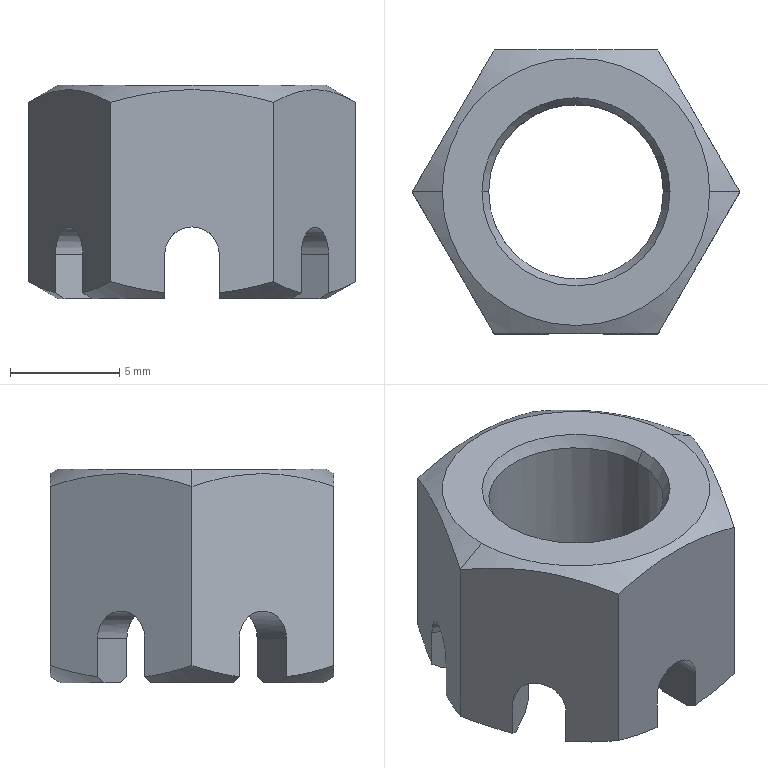Component | SolidWorks | hex slotted nuts style 1-grades c gb-1 | 1 solid | 53 faces | box 15.01 x 13 x 9.8 mm | volume 809 mm3 | plane 25 | cone 18 | cylinder 10 | commonest cylinder face diameters 2.5 x8 8 x2
build123d program:
from build123d import *
from OCP.BRepFilletAPI import BRepFilletAPI_MakeChamfer

# Parameters (mm, degrees)
SKETCH1_R         = 4
BASENUT_DEPTH     = 9.8
ENDCHAMFER_SIZE   = 0.5333
ENDCHAMFER_SIZE2  = 0.3079
SLOT_DEPTH        = 14.951
SLOTPATTERN_COUNT = 3


with BuildPart() as part:
    # Sketch1 → BaseNut (new body)
    with BuildSketch(Plane.XY):
        Polygon((3.753, -6.5), (7.506, 0), (3.753, 6.5), (-3.753, 6.5), (-7.506, 0), (-3.753, -6.5), align=None)
        Circle(SKETCH1_R, mode=Mode.SUBTRACT)
    extrude(amount=-BASENUT_DEPTH)

    # Sketch2 → Double-Chamfer (revolve, cut)
    with BuildSketch(Plane(origin=(0, 0, 0), x_dir=(1, 0, 0), z_dir=(0, 1, 0))):
        Polygon((-7.506, 9.8), (-6.125, 9.8), (-7.506, 9.003), align=None)
        Polygon((-7.506, 0.7971), (-7.506, 0), (-6.125, 0), align=None)
    revolve(axis=Axis((0, 0, -3.376), (0, 0, 1)), mode=Mode.SUBTRACT)

    # EndChamfer: one chamfer whose edges measure the first distance from different faces: ONE call of the kernel's chamfer builder (chamfer() names one face for all edges)
    endchamfer_edges_1 = [part.edges().sort_by_distance(p)[0] for p in [
        (-4, 0, -9.8),
    ]]
    endchamfer_side_1 = [part.faces().sort_by_distance(p)[0] for p in [
        (-4, 0, -4.9),
    ]]
    endchamfer_edges_2 = [part.edges().sort_by_distance(p)[0] for p in [
        (-4, 0, 0),
    ]]
    endchamfer_side_2 = [part.faces().sort_by_distance(p)[0] for p in [
        (5.952, 0, 0),
    ]]
    endchamfer = BRepFilletAPI_MakeChamfer(part.part.solid().wrapped)
    for e in endchamfer_edges_1:
        endchamfer.Add(ENDCHAMFER_SIZE, ENDCHAMFER_SIZE2, e.wrapped, endchamfer_side_1[0].wrapped)  # the first distance lies on this face
    for e in endchamfer_edges_2:
        endchamfer.Add(ENDCHAMFER_SIZE, ENDCHAMFER_SIZE2, e.wrapped, endchamfer_side_2[0].wrapped)  # the first distance lies on this face
    add(Compound.cast(endchamfer.Shape()), mode=Mode.REPLACE)

    # Sketch3 → Slot (cut, symmetric)
    with BuildSketch(Plane(origin=(0, 0, 0), x_dir=(1, 0, 0), z_dir=(0, 1, 0))):
        with BuildLine():
            Line((-1.25, -36.283), (-1.25, 0))
            Line((-1.25, 0), (-1.25, 2.05))
            ThreePointArc((-1.25, 2.05), (0, 3.3), (1.25, 2.05))
            Line((1.25, 2.05), (1.25, 0))
            Line((1.25, 0), (1.25, -36.283))
            Line((1.25, -36.283), (1.25, -108.849))
            Line((1.25, -108.849), (-1.25, -108.849))
            Line((-1.25, -108.849), (-1.25, -36.283))
        make_face()
    slot = extrude(amount=SLOT_DEPTH, both=True, mode=Mode.SUBTRACT)

    # SlotPattern: Slot ×3 about axis
    slotpattern_axis = Axis((0, 0, -3.376), (0, 0, 1))
    for i in range(1, SLOTPATTERN_COUNT):
        add(slot.rotate(slotpattern_axis, i * 360 / SLOTPATTERN_COUNT), mode=Mode.SUBTRACT)


solid = part.part

# Placed as in the assembly
solid = solid.moved(Location((0, 14, -44.4), (180, 0, 0)))